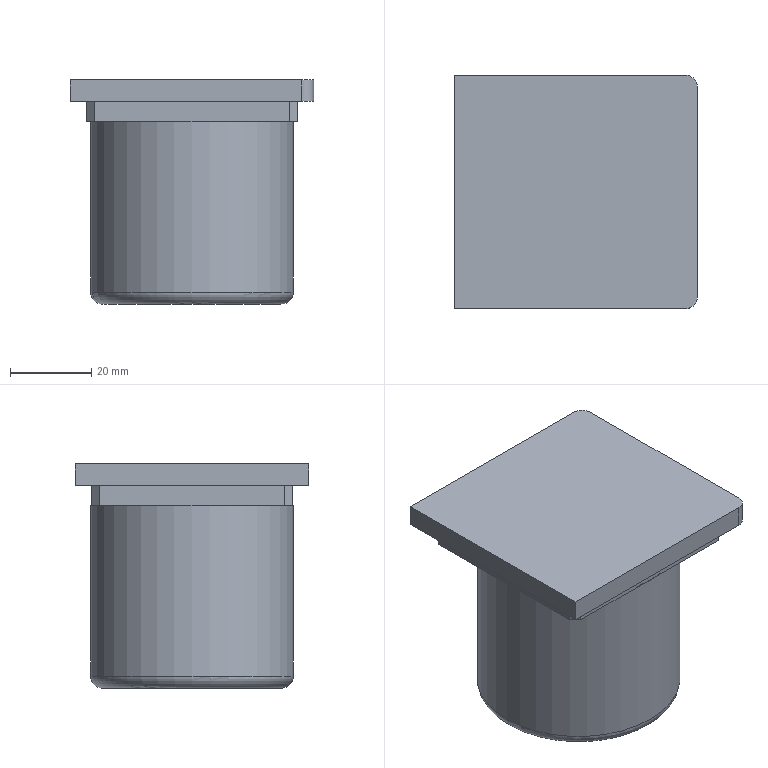Component | NX | MOTOR | 3 solids | 22 faces | volume 119377 mm3 | plane 18 | cylinder 3 | torus 1 | commonest cylinder face diameters 6 x2 50 x1